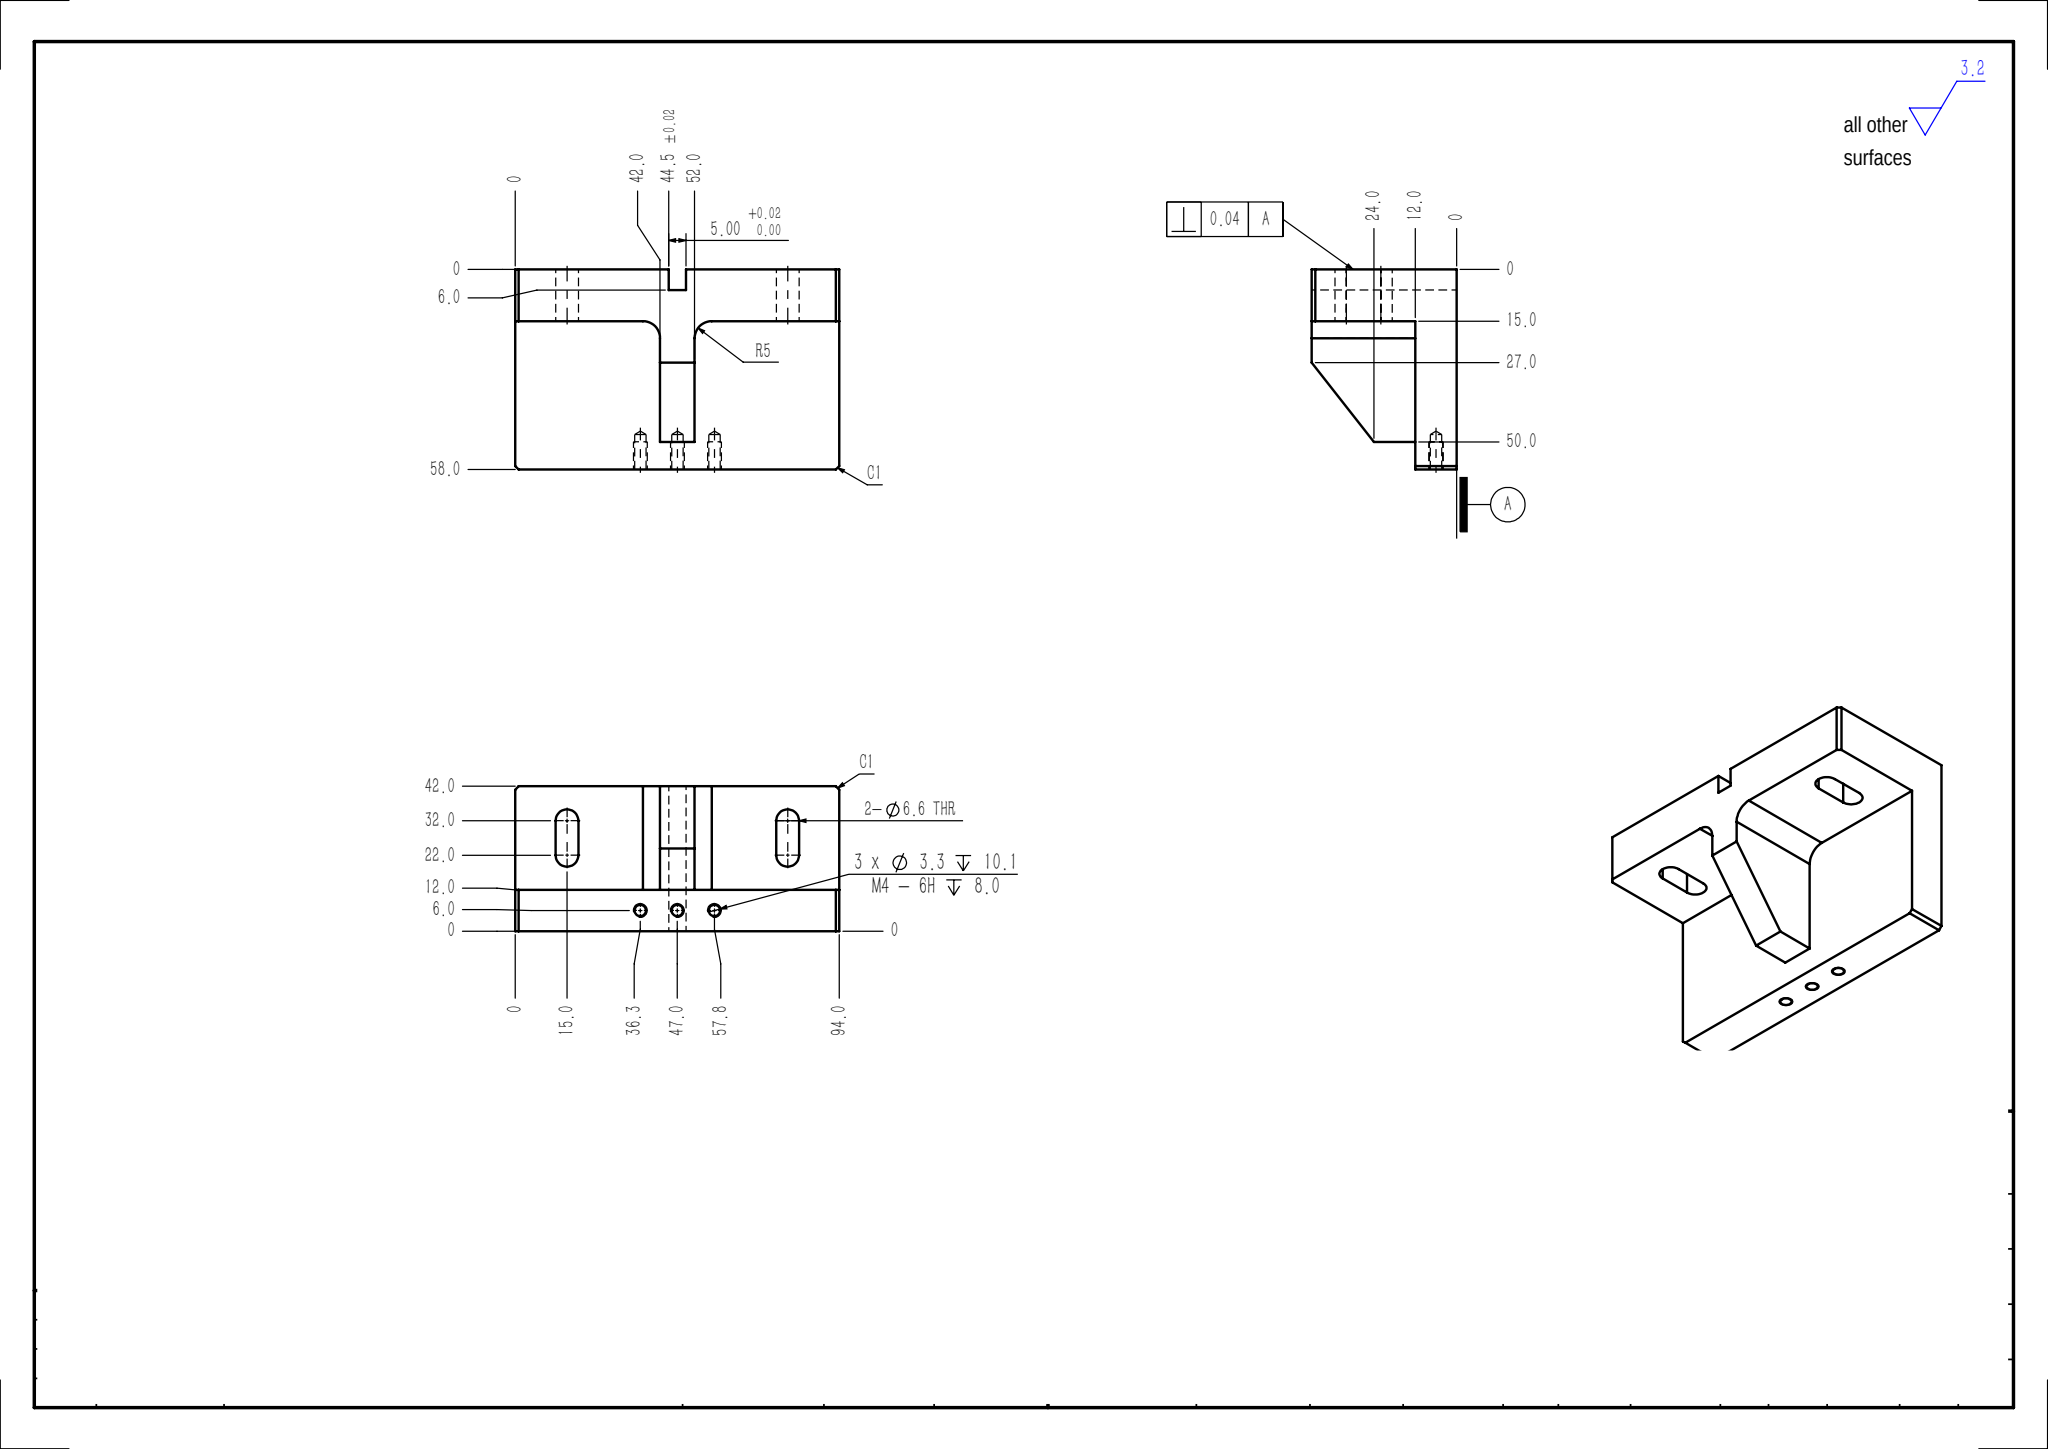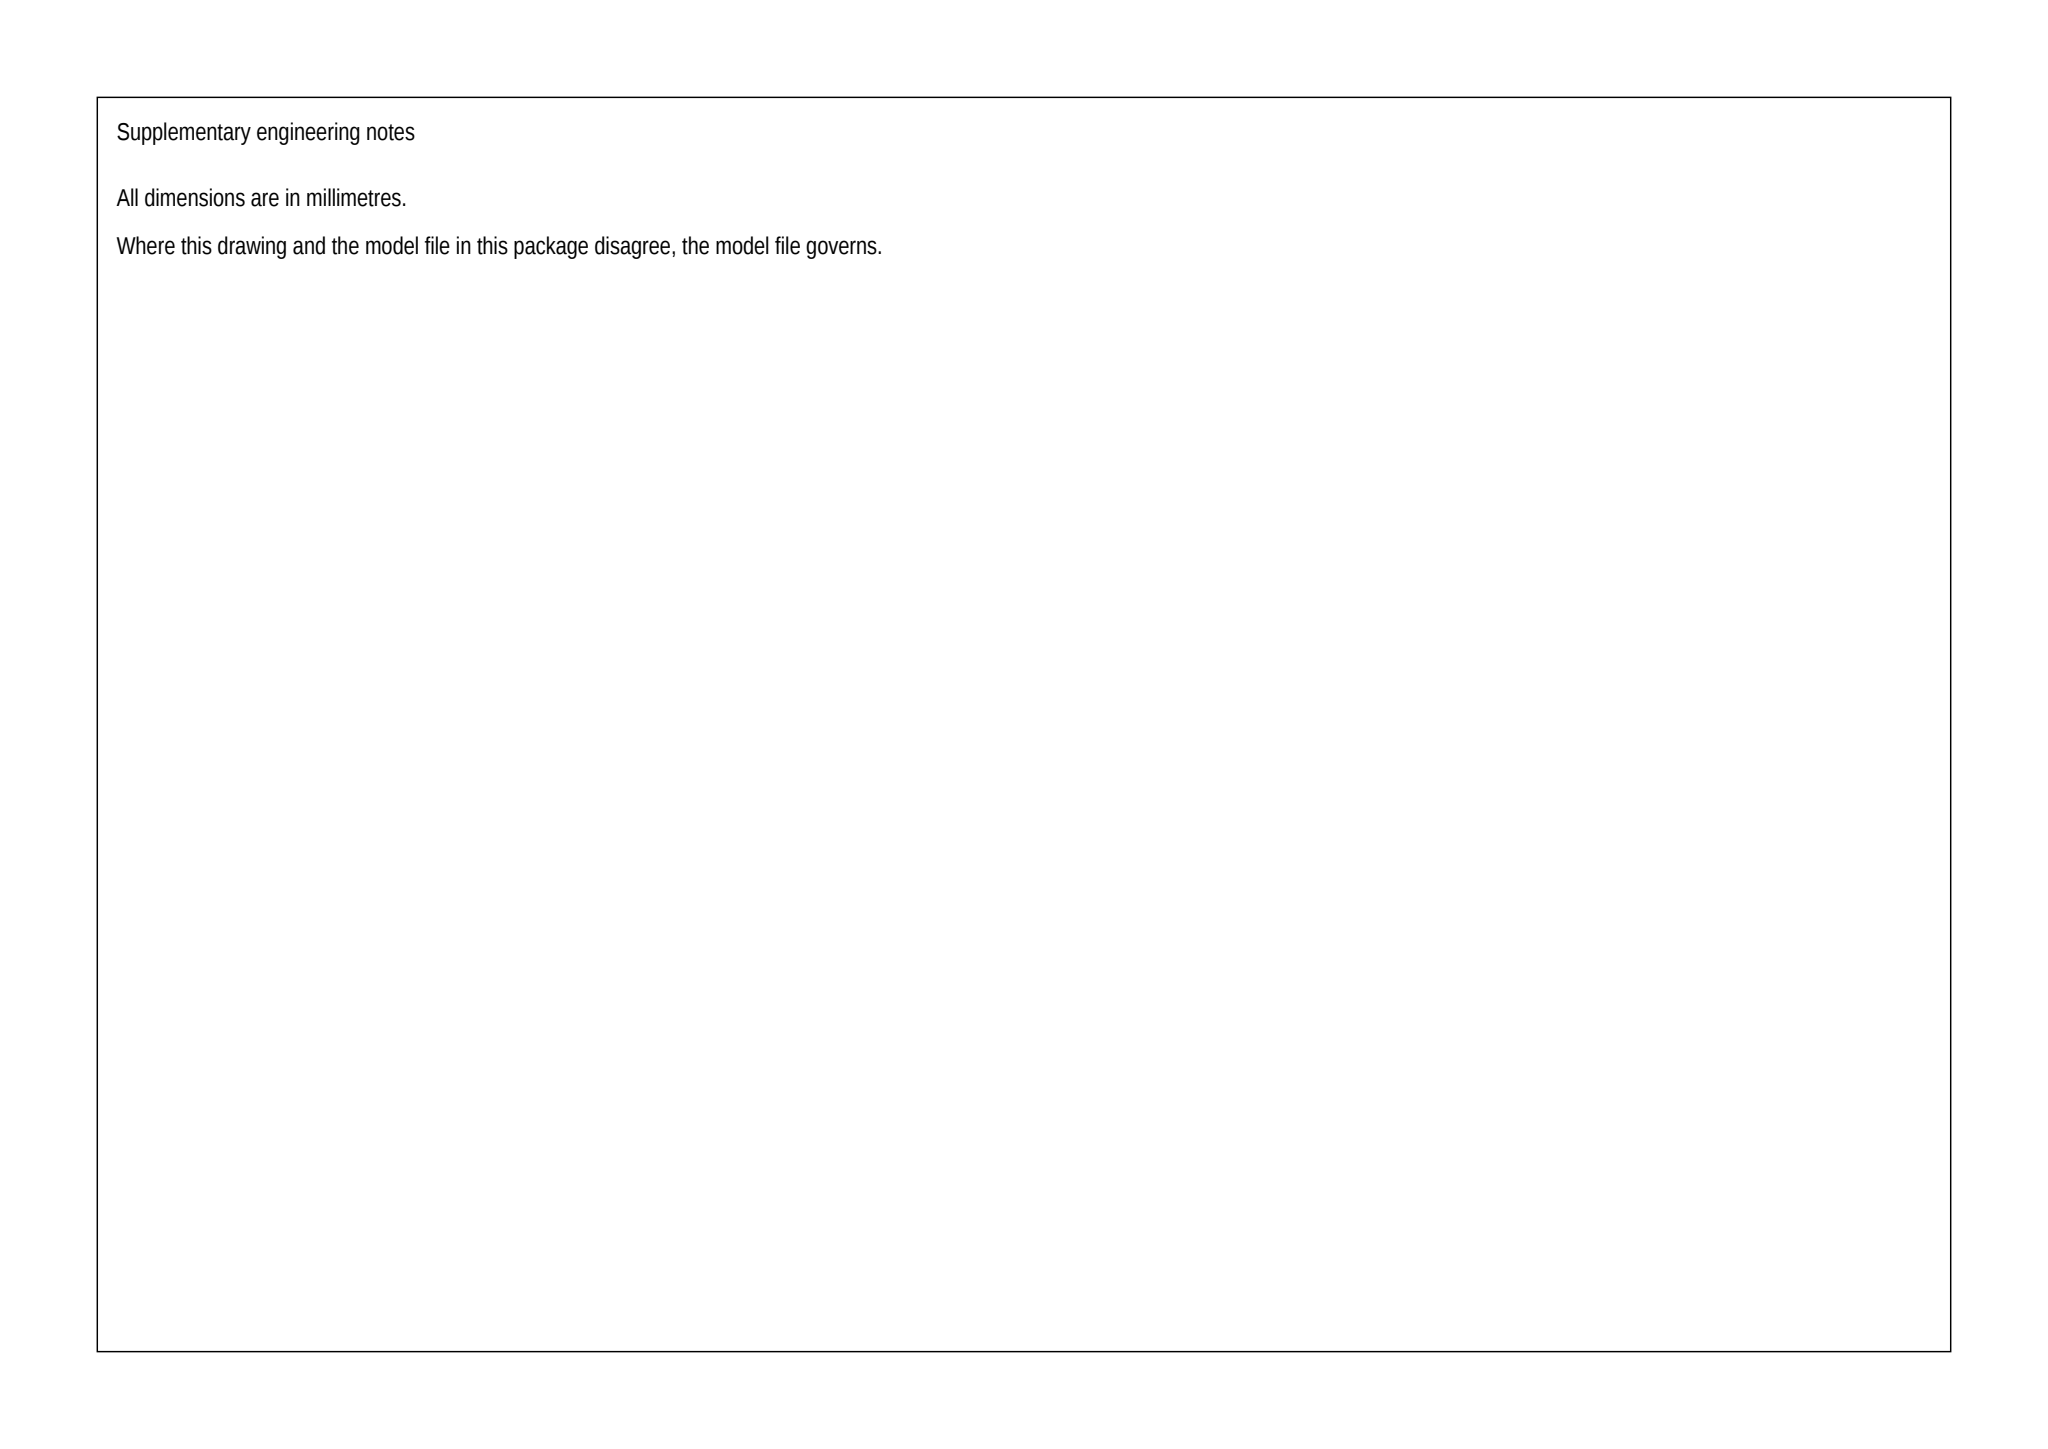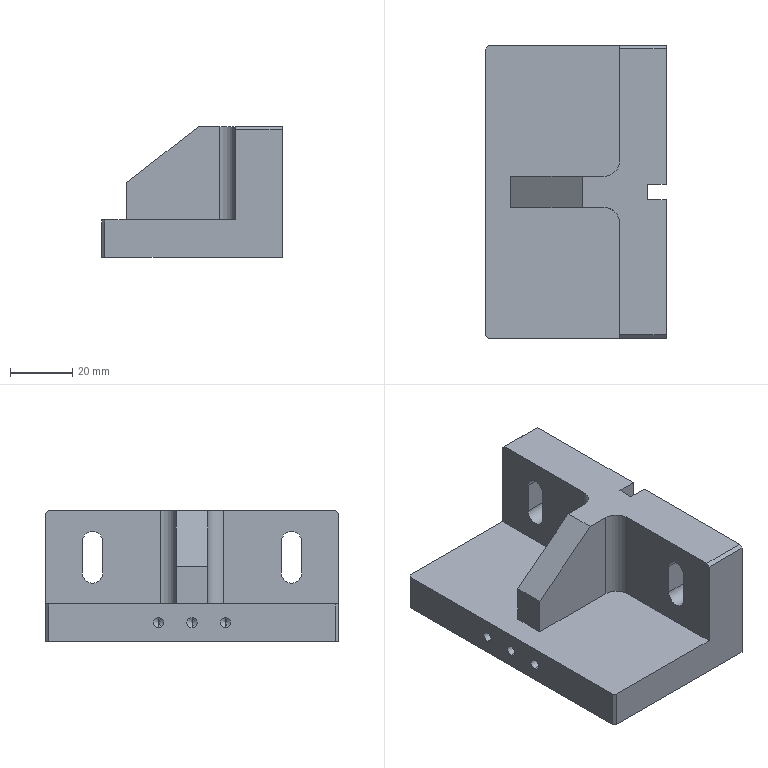Part | SolidWorks | mm | 1 solid | 43 faces | box 58 x 94 x 42 mm | volume 111915 mm3 | plane 25 | cylinder 12 | cone 6 | commonest cylinder face diameters 3.3 x6 6.6 x4 10 x2
build123d program:
from build123d import *

# Parameters (mm, degrees)
SKETCH1_W             = 58
SKETCH1_H             = 94
BOSS_EXTRUDE1_DEPTH   = 12
SKETCH2_W             = 15
SKETCH2_H             = 94
BOSS_EXTRUDE2_DEPTH   = 30
SKETCH3_W             = 84
SKETCH3_H             = 5
CUT_EXTRUDE1_DEPTH    = 6
CUT_EXTRUDE2_DEPTH    = 77.302
BOSS_EXTRUDE3_DEPTH   = 5
FILLET1_R             = 5
CHAMFER1_SIZE         = 1
M4_TAPPED_HOLE1_D     = 3.3
M4_TAPPED_HOLE1_DEPTH = 10.1
M4_TAPPED_HOLE1_TIP   = 0.9914


with BuildPart() as part:
    # Sketch1 → Boss-Extrude1 (new body)
    with BuildSketch(Plane.XY):
        Rectangle(SKETCH1_W, SKETCH1_H)
    extrude(amount=BOSS_EXTRUDE1_DEPTH)

    # Sketch2 → Boss-Extrude2 (add)
    with BuildSketch(Plane.XY.offset(12)):
        with Locations((21.5, 0)):
            Rectangle(SKETCH2_W, SKETCH2_H)
    extrude(amount=BOSS_EXTRUDE2_DEPTH)

    # Sketch3 → Cut-Extrude1 (cut)
    with BuildSketch(Plane(origin=(29, 0, 0), x_dir=(0, 0, -1), z_dir=(1, 0, 0))):
        Rectangle(SKETCH3_W, SKETCH3_H)
    extrude(amount=-CUT_EXTRUDE1_DEPTH, mode=Mode.SUBTRACT)

    # Sketch4 → Cut-Extrude2 (cut, through all)
    with BuildSketch(Plane.ZY.offset(-14)):
        with BuildLine():
            Line((32, 28.7), (22, 28.7))
            ThreePointArc((22, 28.7), (18.7, 32), (22, 35.3))
            Line((22, 35.3), (32, 35.3))
            ThreePointArc((32, 35.3), (35.3, 32), (32, 28.7))
        make_face()
        with BuildLine():
            Line((32, -35.3), (22, -35.3))
            ThreePointArc((22, -35.3), (18.7, -32), (22, -28.7))
            Line((22, -28.7), (32, -28.7))
            ThreePointArc((32, -28.7), (35.3, -32), (32, -35.3))
        make_face()
    extrude(amount=-CUT_EXTRUDE2_DEPTH, mode=Mode.SUBTRACT)

    # Sketch19 → Boss-Extrude3 (add, symmetric)
    with BuildSketch(Plane(origin=(0, 0, 0), x_dir=(1, 0, 0), z_dir=(0, 1, 0))):
        Polygon((-21, -12), (-21, -24), (2, -42), (14, -42), (14, -12), align=None)
    extrude(amount=BOSS_EXTRUDE3_DEPTH, both=True)

    # Fillet1
    fillet1_edges = [part.edges().sort_by_distance(p)[0] for p in [
        (14, -5, 27),
        (14, 5, 27),
    ]]
    fillet(fillet1_edges, radius=FILLET1_R)

    # Chamfer1
    chamfer1_edges = [part.edges().sort_by_distance(p)[0] for p in [
        (21.5, 47, 42),
        (21.5, -47, 42),
        (-29, -47, 6),
        (-29, 47, 6),
    ]]
    chamfer(chamfer1_edges, length=CHAMFER1_SIZE)

    # M4 Tapped Hole1
    with Locations(Plane.ZY.offset(29)):
        with Locations((6, -10.75), (6, 10.75), (6, 0)):
            Hole(M4_TAPPED_HOLE1_D / 2, depth=M4_TAPPED_HOLE1_DEPTH)
            with Locations((0, 0, -(M4_TAPPED_HOLE1_DEPTH + M4_TAPPED_HOLE1_TIP / 2))):  # 118° drill point
                Cone(0, M4_TAPPED_HOLE1_D / 2, M4_TAPPED_HOLE1_TIP, mode=Mode.SUBTRACT)


solid = part.part